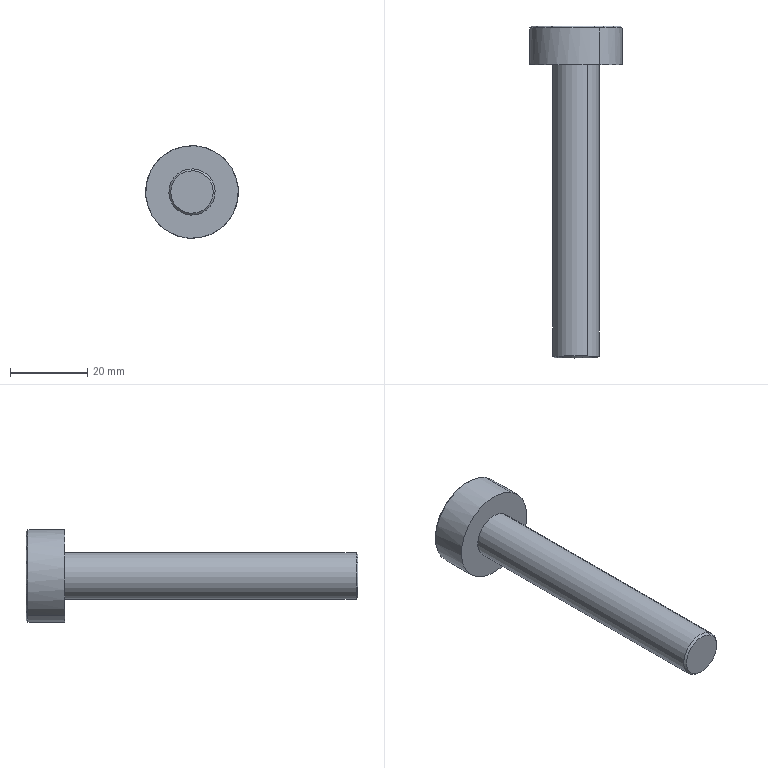Component | SolidWorks | DirectPressureVerticalSeal-1_Pin-1 | 1 solid | 11 faces | box 24 x 86 x 24 mm | volume 13105 mm3 | cylinder 4 | cone 4 | plane 3 | commonest cylinder face diameters 12 x2 24 x2
STEP:
#1=COLOUR_RGB('',0.7922,0.8196,0.9333);
#2=FILL_AREA_STYLE_COLOUR('',#1);
#3=FILL_AREA_STYLE('',(#2));
#4=SURFACE_STYLE_FILL_AREA(#3);
#5=SURFACE_SIDE_STYLE('',(#4));
#6=SURFACE_STYLE_USAGE(.BOTH.,#5);
#7=PRESENTATION_STYLE_ASSIGNMENT((#6));
#8=CARTESIAN_POINT('',(-18.333,8.243,11.561));
#9=VERTEX_POINT('',#8);
#10=CARTESIAN_POINT('',(-18.576,8.243,11.156));
#11=VERTEX_POINT('',#10);
#12=CARTESIAN_POINT('',(-18.455,8.243,11.358));
#13=DIRECTION('',(0.,1.,0.));
#14=DIRECTION('',(0.5151,0.,0.8572));
#15=AXIS2_PLACEMENT_3D('',#12,#13,#14);
#16=CIRCLE('',#15,0.2362);
#17=EDGE_CURVE('',#9,#11,#16,.T.);
#18=ORIENTED_EDGE('',*,*,#17,.T.);
#19=CARTESIAN_POINT('',(-18.576,11.215,11.156));
#20=VERTEX_POINT('',#19);
#21=CARTESIAN_POINT('',(-18.576,11.609,11.156));
#22=DIRECTION('',(0.,1.,0.));
#23=VECTOR('',#22,39.37);
#24=LINE('',#21,#23);
#25=EDGE_CURVE('',#11,#20,#24,.T.);
#26=ORIENTED_EDGE('',*,*,#25,.T.);
#27=CARTESIAN_POINT('',(-18.333,11.215,11.561));
#28=VERTEX_POINT('',#27);
#29=CARTESIAN_POINT('',(-18.455,11.215,11.358));
#30=DIRECTION('',(-0.,-1.,-0.));
#31=DIRECTION('',(0.5151,0.,0.8572));
#32=AXIS2_PLACEMENT_3D('',#29,#30,#31);
#33=CIRCLE('',#32,0.2362);
#34=EDGE_CURVE('',#20,#28,#33,.T.);
#35=ORIENTED_EDGE('',*,*,#34,.T.);
#36=CARTESIAN_POINT('',(-18.333,11.609,11.561));
#37=DIRECTION('',(0.,1.,0.));
#38=VECTOR('',#37,39.37);
#39=LINE('',#36,#38);
#40=EDGE_CURVE('',#9,#28,#39,.T.);
#41=ORIENTED_EDGE('',*,*,#40,.F.);
#42=EDGE_LOOP('',(#18,#26,#35,#41));
#43=FACE_OUTER_BOUND('',#42,.T.);
#44=CARTESIAN_POINT('',(-18.455,11.609,11.358));
#45=DIRECTION('',(0.,1.,0.));
#46=DIRECTION('',(0.5151,0.,0.8572));
#47=AXIS2_PLACEMENT_3D('',#44,#45,#46);
#48=CYLINDRICAL_SURFACE('',#47,0.2362);
#49=ADVANCED_FACE('',(#43),#48,.T.);
#50=CARTESIAN_POINT('',(-18.343,8.223,11.544));
#51=VERTEX_POINT('',#50);
#52=CARTESIAN_POINT('',(-18.566,8.223,11.173));
#53=VERTEX_POINT('',#52);
#54=CARTESIAN_POINT('',(-18.455,8.223,11.358));
#55=DIRECTION('',(0.,1.,0.));
#56=DIRECTION('',(0.5151,0.,0.8572));
#57=AXIS2_PLACEMENT_3D('',#54,#55,#56);
#58=CIRCLE('',#57,0.2165);
#59=EDGE_CURVE('',#51,#53,#58,.T.);
#60=ORIENTED_EDGE('',*,*,#59,.T.);
#61=CARTESIAN_POINT('',(-18.576,8.243,11.156));
#62=DIRECTION('',(-0.3642,0.7071,-0.6061));
#63=VECTOR('',#62,39.37);
#64=LINE('',#61,#63);
#65=EDGE_CURVE('',#53,#11,#64,.T.);
#66=ORIENTED_EDGE('',*,*,#65,.T.);
#67=ORIENTED_EDGE('',*,*,#17,.F.);
#68=CARTESIAN_POINT('',(-18.333,8.243,11.561));
#69=DIRECTION('',(0.3642,0.7071,0.6061));
#70=VECTOR('',#69,39.37);
#71=LINE('',#68,#70);
#72=EDGE_CURVE('',#51,#9,#71,.T.);
#73=ORIENTED_EDGE('',*,*,#72,.F.);
#74=EDGE_LOOP('',(#60,#66,#67,#73));
#75=FACE_OUTER_BOUND('',#74,.T.);
#76=CARTESIAN_POINT('',(-18.455,8.243,11.358));
#77=DIRECTION('',(0.,1.,0.));
#78=DIRECTION('',(0.5151,0.,0.8572));
#79=AXIS2_PLACEMENT_3D('',#76,#77,#78);
#80=CONICAL_SURFACE('',#79,0.2362,0.7854);
#81=ADVANCED_FACE('',(#75),#80,.T.);
#82=CARTESIAN_POINT('',(-18.211,11.215,11.763));
#83=VERTEX_POINT('',#82);
#84=CARTESIAN_POINT('',(-18.698,11.215,10.953));
#85=VERTEX_POINT('',#84);
#86=CARTESIAN_POINT('',(-18.455,11.215,11.358));
#87=DIRECTION('',(0.,1.,0.));
#88=DIRECTION('',(0.5151,0.,0.8572));
#89=AXIS2_PLACEMENT_3D('',#86,#87,#88);
#90=CIRCLE('',#89,0.4724);
#91=EDGE_CURVE('',#83,#85,#90,.T.);
#92=ORIENTED_EDGE('',*,*,#91,.T.);
#93=CARTESIAN_POINT('',(-18.698,11.59,10.953));
#94=VERTEX_POINT('',#93);
#95=CARTESIAN_POINT('',(-18.698,11.609,10.953));
#96=DIRECTION('',(0.,1.,0.));
#97=VECTOR('',#96,39.37);
#98=LINE('',#95,#97);
#99=EDGE_CURVE('',#85,#94,#98,.T.);
#100=ORIENTED_EDGE('',*,*,#99,.T.);
#101=CARTESIAN_POINT('',(-18.05,11.59,11.115));
#102=VERTEX_POINT('',#101);
#103=CARTESIAN_POINT('',(-18.455,11.59,11.358));
#104=DIRECTION('',(-0.,-1.,-0.));
#105=DIRECTION('',(0.5151,0.,0.8572));
#106=AXIS2_PLACEMENT_3D('',#103,#104,#105);
#107=CIRCLE('',#106,0.4724);
#108=EDGE_CURVE('',#94,#102,#107,.T.);
#109=ORIENTED_EDGE('',*,*,#108,.T.);
#110=CARTESIAN_POINT('',(-18.211,11.59,11.763));
#111=VERTEX_POINT('',#110);
#112=CARTESIAN_POINT('',(-18.455,11.59,11.358));
#113=DIRECTION('',(-0.,-1.,-0.));
#114=DIRECTION('',(0.5151,0.,0.8572));
#115=AXIS2_PLACEMENT_3D('',#112,#113,#114);
#116=CIRCLE('',#115,0.4724);
#117=EDGE_CURVE('',#102,#111,#116,.T.);
#118=ORIENTED_EDGE('',*,*,#117,.T.);
#119=CARTESIAN_POINT('',(-18.211,11.609,11.763));
#120=DIRECTION('',(0.,1.,0.));
#121=VECTOR('',#120,39.37);
#122=LINE('',#119,#121);
#123=EDGE_CURVE('',#83,#111,#122,.T.);
#124=ORIENTED_EDGE('',*,*,#123,.F.);
#125=EDGE_LOOP('',(#92,#100,#109,#118,#124));
#126=FACE_OUTER_BOUND('',#125,.T.);
#127=CARTESIAN_POINT('',(-18.455,11.609,11.358));
#128=DIRECTION('',(0.,1.,0.));
#129=DIRECTION('',(0.5151,0.,0.8572));
#130=AXIS2_PLACEMENT_3D('',#127,#128,#129);
#131=CYLINDRICAL_SURFACE('',#130,0.4724);
#132=ADVANCED_FACE('',(#126),#131,.T.);
#133=CARTESIAN_POINT('',(-18.066,11.609,11.125));
#134=VERTEX_POINT('',#133);
#135=CARTESIAN_POINT('',(-18.843,11.609,11.591));
#136=VERTEX_POINT('',#135);
#137=CARTESIAN_POINT('',(-18.455,11.609,11.358));
#138=DIRECTION('',(-0.,-1.,-0.));
#139=DIRECTION('',(0.8572,0.,-0.5151));
#140=AXIS2_PLACEMENT_3D('',#137,#138,#139);
#141=CIRCLE('',#140,0.4528);
#142=EDGE_CURVE('',#134,#136,#141,.T.);
#143=ORIENTED_EDGE('',*,*,#142,.T.);
#144=CARTESIAN_POINT('',(-18.86,11.59,11.602));
#145=VERTEX_POINT('',#144);
#146=CARTESIAN_POINT('',(-18.86,11.59,11.602));
#147=DIRECTION('',(-0.6061,-0.7071,0.3642));
#148=VECTOR('',#147,39.37);
#149=LINE('',#146,#148);
#150=EDGE_CURVE('',#136,#145,#149,.T.);
#151=ORIENTED_EDGE('',*,*,#150,.T.);
#152=CARTESIAN_POINT('',(-18.455,11.59,11.358));
#153=DIRECTION('',(-0.,-1.,-0.));
#154=DIRECTION('',(0.5151,0.,0.8572));
#155=AXIS2_PLACEMENT_3D('',#152,#153,#154);
#156=CIRCLE('',#155,0.4724);
#157=EDGE_CURVE('',#111,#145,#156,.T.);
#158=ORIENTED_EDGE('',*,*,#157,.F.);
#159=ORIENTED_EDGE('',*,*,#117,.F.);
#160=CARTESIAN_POINT('',(-18.05,11.59,11.115));
#161=DIRECTION('',(0.6061,-0.7071,-0.3642));
#162=VECTOR('',#161,39.37);
#163=LINE('',#160,#162);
#164=EDGE_CURVE('',#134,#102,#163,.T.);
#165=ORIENTED_EDGE('',*,*,#164,.F.);
#166=EDGE_LOOP('',(#143,#151,#158,#159,#165));
#167=FACE_OUTER_BOUND('',#166,.T.);
#168=CARTESIAN_POINT('',(-18.455,11.59,11.358));
#169=DIRECTION('',(-0.,-1.,-0.));
#170=DIRECTION('',(0.8572,0.,-0.5151));
#171=AXIS2_PLACEMENT_3D('',#168,#169,#170);
#172=CONICAL_SURFACE('',#171,0.4724,0.7854);
#173=ADVANCED_FACE('',(#167),#172,.T.);
#174=ORIENTED_EDGE('',*,*,#25,.F.);
#175=CARTESIAN_POINT('',(-18.455,8.243,11.358));
#176=DIRECTION('',(0.,1.,0.));
#177=DIRECTION('',(0.5151,0.,0.8572));
#178=AXIS2_PLACEMENT_3D('',#175,#176,#177);
#179=CIRCLE('',#178,0.2362);
#180=EDGE_CURVE('',#11,#9,#179,.T.);
#181=ORIENTED_EDGE('',*,*,#180,.T.);
#182=ORIENTED_EDGE('',*,*,#40,.T.);
#183=CARTESIAN_POINT('',(-18.455,11.215,11.358));
#184=DIRECTION('',(-0.,-1.,-0.));
#185=DIRECTION('',(0.5151,0.,0.8572));
#186=AXIS2_PLACEMENT_3D('',#183,#184,#185);
#187=CIRCLE('',#186,0.2362);
#188=EDGE_CURVE('',#28,#20,#187,.T.);
#189=ORIENTED_EDGE('',*,*,#188,.T.);
#190=EDGE_LOOP('',(#174,#181,#182,#189));
#191=FACE_OUTER_BOUND('',#190,.T.);
#192=CARTESIAN_POINT('',(-18.455,11.609,11.358));
#193=DIRECTION('',(0.,1.,0.));
#194=DIRECTION('',(0.5151,0.,0.8572));
#195=AXIS2_PLACEMENT_3D('',#192,#193,#194);
#196=CYLINDRICAL_SURFACE('',#195,0.2362);
#197=ADVANCED_FACE('',(#191),#196,.T.);
#198=ORIENTED_EDGE('',*,*,#91,.F.);
#199=CARTESIAN_POINT('',(-18.455,11.215,11.358));
#200=DIRECTION('',(0.,1.,0.));
#201=DIRECTION('',(0.5151,0.,0.8572));
#202=AXIS2_PLACEMENT_3D('',#199,#200,#201);
#203=CIRCLE('',#202,0.4724);
#204=EDGE_CURVE('',#85,#83,#203,.T.);
#205=ORIENTED_EDGE('',*,*,#204,.F.);
#206=EDGE_LOOP('',(#198,#205));
#207=FACE_OUTER_BOUND('',#206,.T.);
#208=ORIENTED_EDGE('',*,*,#188,.F.);
#209=ORIENTED_EDGE('',*,*,#34,.F.);
#210=EDGE_LOOP('',(#208,#209));
#211=FACE_BOUND('',#210,.T.);
#212=CARTESIAN_POINT('',(-18.252,11.215,11.237));
#213=DIRECTION('',(0.,1.,0.));
#214=DIRECTION('',(0.5151,-0.,0.8572));
#215=AXIS2_PLACEMENT_3D('',#212,#213,#214);
#216=PLANE('',#215);
#217=ADVANCED_FACE('',(#207,#211),#216,.F.);
#218=ORIENTED_EDGE('',*,*,#65,.F.);
#219=CARTESIAN_POINT('',(-18.455,8.223,11.358));
#220=DIRECTION('',(0.,1.,0.));
#221=DIRECTION('',(0.5151,0.,0.8572));
#222=AXIS2_PLACEMENT_3D('',#219,#220,#221);
#223=CIRCLE('',#222,0.2165);
#224=EDGE_CURVE('',#53,#51,#223,.T.);
#225=ORIENTED_EDGE('',*,*,#224,.T.);
#226=ORIENTED_EDGE('',*,*,#72,.T.);
#227=ORIENTED_EDGE('',*,*,#180,.F.);
#228=EDGE_LOOP('',(#218,#225,#226,#227));
#229=FACE_OUTER_BOUND('',#228,.T.);
#230=CARTESIAN_POINT('',(-18.455,8.243,11.358));
#231=DIRECTION('',(0.,1.,0.));
#232=DIRECTION('',(0.5151,0.,0.8572));
#233=AXIS2_PLACEMENT_3D('',#230,#231,#232);
#234=CONICAL_SURFACE('',#233,0.2362,0.7854);
#235=ADVANCED_FACE('',(#229),#234,.T.);
#236=ORIENTED_EDGE('',*,*,#99,.F.);
#237=ORIENTED_EDGE('',*,*,#204,.T.);
#238=ORIENTED_EDGE('',*,*,#123,.T.);
#239=ORIENTED_EDGE('',*,*,#157,.T.);
#240=CARTESIAN_POINT('',(-18.455,11.59,11.358));
#241=DIRECTION('',(-0.,-1.,-0.));
#242=DIRECTION('',(0.5151,0.,0.8572));
#243=AXIS2_PLACEMENT_3D('',#240,#241,#242);
#244=CIRCLE('',#243,0.4724);
#245=EDGE_CURVE('',#145,#94,#244,.T.);
#246=ORIENTED_EDGE('',*,*,#245,.T.);
#247=EDGE_LOOP('',(#236,#237,#238,#239,#246));
#248=FACE_OUTER_BOUND('',#247,.T.);
#249=CARTESIAN_POINT('',(-18.455,11.609,11.358));
#250=DIRECTION('',(0.,1.,0.));
#251=DIRECTION('',(0.5151,0.,0.8572));
#252=AXIS2_PLACEMENT_3D('',#249,#250,#251);
#253=CYLINDRICAL_SURFACE('',#252,0.4724);
#254=ADVANCED_FACE('',(#248),#253,.T.);
#255=ORIENTED_EDGE('',*,*,#59,.F.);
#256=ORIENTED_EDGE('',*,*,#224,.F.);
#257=EDGE_LOOP('',(#255,#256));
#258=FACE_OUTER_BOUND('',#257,.T.);
#259=CARTESIAN_POINT('',(-18.455,8.223,11.358));
#260=DIRECTION('',(0.,1.,0.));
#261=DIRECTION('',(0.5151,-0.,0.8572));
#262=AXIS2_PLACEMENT_3D('',#259,#260,#261);
#263=PLANE('',#262);
#264=ADVANCED_FACE('',(#258),#263,.F.);
#265=ORIENTED_EDGE('',*,*,#150,.F.);
#266=CARTESIAN_POINT('',(-18.455,11.609,11.358));
#267=DIRECTION('',(-0.,-1.,-0.));
#268=DIRECTION('',(0.8572,0.,-0.5151));
#269=AXIS2_PLACEMENT_3D('',#266,#267,#268);
#270=CIRCLE('',#269,0.4528);
#271=EDGE_CURVE('',#136,#134,#270,.T.);
#272=ORIENTED_EDGE('',*,*,#271,.T.);
#273=ORIENTED_EDGE('',*,*,#164,.T.);
#274=ORIENTED_EDGE('',*,*,#108,.F.);
#275=ORIENTED_EDGE('',*,*,#245,.F.);
#276=EDGE_LOOP('',(#265,#272,#273,#274,#275));
#277=FACE_OUTER_BOUND('',#276,.T.);
#278=CARTESIAN_POINT('',(-18.455,11.59,11.358));
#279=DIRECTION('',(-0.,-1.,-0.));
#280=DIRECTION('',(0.8572,0.,-0.5151));
#281=AXIS2_PLACEMENT_3D('',#278,#279,#280);
#282=CONICAL_SURFACE('',#281,0.4724,0.7854);
#283=ADVANCED_FACE('',(#277),#282,.T.);
#284=ORIENTED_EDGE('',*,*,#142,.F.);
#285=ORIENTED_EDGE('',*,*,#271,.F.);
#286=EDGE_LOOP('',(#284,#285));
#287=FACE_OUTER_BOUND('',#286,.T.);
#288=CARTESIAN_POINT('',(-18.066,11.609,11.125));
#289=DIRECTION('',(-0.,-1.,-0.));
#290=DIRECTION('',(-0.5151,0.,-0.8572));
#291=AXIS2_PLACEMENT_3D('',#288,#289,#290);
#292=PLANE('',#291);
#293=ADVANCED_FACE('',(#287),#292,.F.);
#294=CLOSED_SHELL('',(#49,#81,#132,#173,#197,#217,#235,#254,#264,#283,#293));
#295=MANIFOLD_SOLID_BREP('',#294);
#296=STYLED_ITEM('',(#7),#295);
#297=(LENGTH_UNIT()NAMED_UNIT(*)SI_UNIT($,.METRE.));
#298=LENGTH_MEASURE_WITH_UNIT(LENGTH_MEASURE(0.0254),#297);
#299=DIMENSIONAL_EXPONENTS(1.,0.,0.,0.,0.,0.,0.);
#300=(CONVERSION_BASED_UNIT('',#298)LENGTH_UNIT()NAMED_UNIT(#299));
#301=UNCERTAINTY_MEASURE_WITH_UNIT(LENGTH_MEASURE(0.00001),#300,'','');
#302=(NAMED_UNIT(*)PLANE_ANGLE_UNIT()SI_UNIT($,.RADIAN.));
#303=(NAMED_UNIT(*)SI_UNIT($,.STERADIAN.)SOLID_ANGLE_UNIT());
#304=(GEOMETRIC_REPRESENTATION_CONTEXT(3)GLOBAL_UNCERTAINTY_ASSIGNED_CONTEXT((#301))GLOBAL_UNIT_ASSIGNED_CONTEXT((#300,#302,#303))REPRESENTATION_CONTEXT('',''));
#305=MECHANICAL_DESIGN_GEOMETRIC_PRESENTATION_REPRESENTATION('',(#296),#304);
#306=PRESENTATION_LAYER_ASSIGNMENT('','',(#296));
#307=CARTESIAN_POINT('',(0.,0.,0.));
#308=DIRECTION('',(0.,0.,1.));
#309=DIRECTION('',(1.,0.,0.));
#310=AXIS2_PLACEMENT_3D('',#307,#308,#309);
#311=(LENGTH_UNIT()NAMED_UNIT(*)SI_UNIT($,.METRE.));
#312=LENGTH_MEASURE_WITH_UNIT(LENGTH_MEASURE(0.0254),#311);
#313=DIMENSIONAL_EXPONENTS(1.,0.,0.,0.,0.,0.,0.);
#314=(CONVERSION_BASED_UNIT('',#312)LENGTH_UNIT()NAMED_UNIT(#313));
#315=UNCERTAINTY_MEASURE_WITH_UNIT(LENGTH_MEASURE(0.00001),#314,'','');
#316=(NAMED_UNIT(*)PLANE_ANGLE_UNIT()SI_UNIT($,.RADIAN.));
#317=(NAMED_UNIT(*)SI_UNIT($,.STERADIAN.)SOLID_ANGLE_UNIT());
#318=(GEOMETRIC_REPRESENTATION_CONTEXT(3)GLOBAL_UNCERTAINTY_ASSIGNED_CONTEXT((#315))GLOBAL_UNIT_ASSIGNED_CONTEXT((#314,#316,#317))REPRESENTATION_CONTEXT('',''));
#319=ADVANCED_BREP_SHAPE_REPRESENTATION('',(#295,#310),#318);